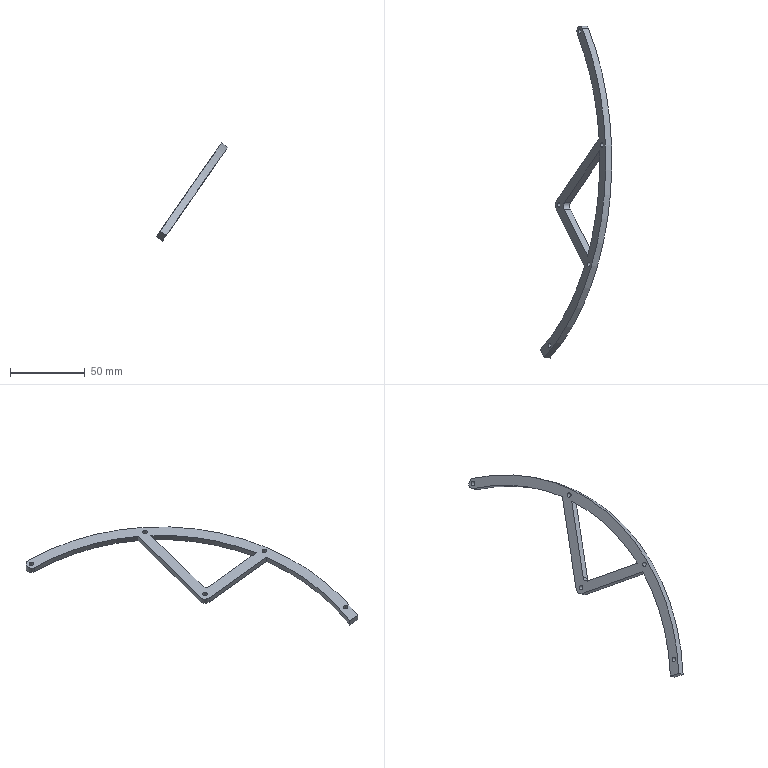Component | NX | LOWER_LEG_2 | 1 solid | 19 faces | volume 12489 mm3 | cylinder 12 | plane 7 | commonest cylinder face diameters 3 x5 300 x3 8.286 x1 7 x1 314 x1 6.571 x1